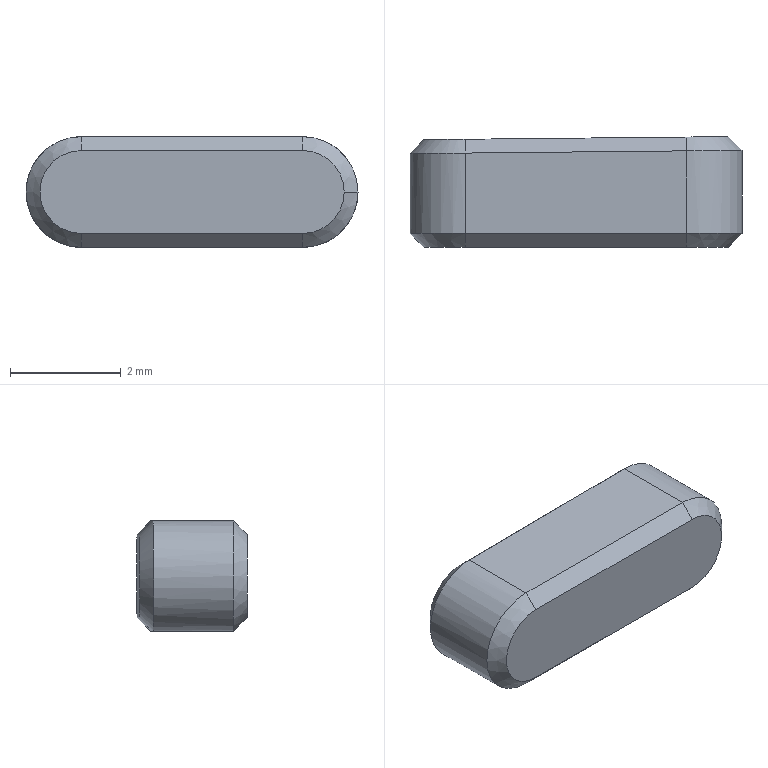Component | SolidWorks | taper keys for general use gb-2 | 1 solid | 16 faces | box 6 x 2 x 2 mm | volume 21 mm3 | plane 8 | cone 3 | cylinder 3 | spline 2 | commonest cylinder face diameters 2 x3
STEP:
#1=COLOUR_RGB('',0.7922,0.8196,0.9333);
#2=FILL_AREA_STYLE_COLOUR('',#1);
#3=FILL_AREA_STYLE('',(#2));
#4=SURFACE_STYLE_FILL_AREA(#3);
#5=SURFACE_SIDE_STYLE('',(#4));
#6=SURFACE_STYLE_USAGE(.BOTH.,#5);
#7=PRESENTATION_STYLE_ASSIGNMENT((#6));
#8=CARTESIAN_POINT('',(15.268,0.851,13.74));
#9=VERTEX_POINT('',#8);
#10=CARTESIAN_POINT('',(15.239,0.851,13.77));
#11=VERTEX_POINT('',#10);
#12=CARTESIAN_POINT('',(15.239,0.851,13.74));
#13=DIRECTION('',(-0.,-1.,0.));
#14=DIRECTION('',(1.,0.,0.));
#15=AXIS2_PLACEMENT_3D('',#12,#13,#14);
#16=CIRCLE('',#15,0.02953);
#17=EDGE_CURVE('',#9,#11,#16,.T.);
#18=ORIENTED_EDGE('',*,*,#17,.F.);
#19=CARTESIAN_POINT('',(15.278,0.8609,13.74));
#20=VERTEX_POINT('',#19);
#21=CARTESIAN_POINT('',(15.268,0.851,13.74));
#22=DIRECTION('',(0.7071,0.7071,-0.));
#23=VECTOR('',#22,39.37);
#24=LINE('',#21,#23);
#25=EDGE_CURVE('',#9,#20,#24,.T.);
#26=ORIENTED_EDGE('',*,*,#25,.T.);
#27=CARTESIAN_POINT('',(15.239,0.8609,13.78));
#28=VERTEX_POINT('',#27);
#29=CARTESIAN_POINT('',(15.239,0.8609,13.74));
#30=DIRECTION('',(0.,1.,-0.));
#31=DIRECTION('',(1.,0.,0.));
#32=AXIS2_PLACEMENT_3D('',#29,#30,#31);
#33=CIRCLE('',#32,0.03937);
#34=EDGE_CURVE('',#28,#20,#33,.T.);
#35=ORIENTED_EDGE('',*,*,#34,.F.);
#36=CARTESIAN_POINT('',(15.239,0.851,13.77));
#37=DIRECTION('',(-0.,0.7071,0.7071));
#38=VECTOR('',#37,39.37);
#39=LINE('',#36,#38);
#40=EDGE_CURVE('',#11,#28,#39,.T.);
#41=ORIENTED_EDGE('',*,*,#40,.F.);
#42=EDGE_LOOP('',(#18,#26,#35,#41));
#43=FACE_OUTER_BOUND('',#42,.T.);
#44=CARTESIAN_POINT('',(15.239,0.851,13.74));
#45=DIRECTION('',(0.,1.,-0.));
#46=DIRECTION('',(1.,0.,0.));
#47=AXIS2_PLACEMENT_3D('',#44,#45,#46);
#48=CONICAL_SURFACE('',#47,0.02953,0.7854);
#49=ADVANCED_FACE('',(#43),#48,.T.);
#50=ORIENTED_EDGE('',*,*,#34,.T.);
#51=CARTESIAN_POINT('',(15.278,0.9198,13.74));
#52=VERTEX_POINT('',#51);
#53=CARTESIAN_POINT('',(15.278,0.851,13.74));
#54=DIRECTION('',(0.,1.,-0.));
#55=VECTOR('',#54,39.37);
#56=LINE('',#53,#55);
#57=EDGE_CURVE('',#20,#52,#56,.T.);
#58=ORIENTED_EDGE('',*,*,#57,.T.);
#59=CARTESIAN_POINT('',(15.239,0.9195,13.78));
#60=VERTEX_POINT('',#59);
#61=CARTESIAN_POINT('',(15.278,0.9198,13.74));
#62=CARTESIAN_POINT('',(15.278,0.9198,13.744));
#63=CARTESIAN_POINT('',(15.277,0.9198,13.748));
#64=CARTESIAN_POINT('',(15.275,0.9198,13.756));
#65=CARTESIAN_POINT('',(15.273,0.9198,13.761));
#66=CARTESIAN_POINT('',(15.266,0.9197,13.769));
#67=CARTESIAN_POINT('',(15.262,0.9197,13.773));
#68=CARTESIAN_POINT('',(15.251,0.9196,13.778));
#69=CARTESIAN_POINT('',(15.245,0.9196,13.78));
#70=CARTESIAN_POINT('',(15.239,0.9195,13.78));
#71=B_SPLINE_CURVE_WITH_KNOTS('',3,(#61,#62,#63,#64,#65,#66,#67,#68,#69,#70),.UNSPECIFIED.,.F.,.F.,(4,2,2,2,4),(0.5,0.625,0.75,0.875,1.),.UNSPECIFIED.);
#72=EDGE_CURVE('',#52,#60,#71,.T.);
#73=ORIENTED_EDGE('',*,*,#72,.T.);
#74=CARTESIAN_POINT('',(15.239,0.851,13.78));
#75=DIRECTION('',(0.,1.,-0.));
#76=VECTOR('',#75,39.37);
#77=LINE('',#74,#76);
#78=EDGE_CURVE('',#28,#60,#77,.T.);
#79=ORIENTED_EDGE('',*,*,#78,.F.);
#80=EDGE_LOOP('',(#50,#58,#73,#79));
#81=FACE_OUTER_BOUND('',#80,.T.);
#82=CARTESIAN_POINT('',(15.239,0.851,13.74));
#83=DIRECTION('',(0.,1.,-0.));
#84=DIRECTION('',(1.,0.,0.));
#85=AXIS2_PLACEMENT_3D('',#82,#83,#84);
#86=CYLINDRICAL_SURFACE('',#85,0.03937);
#87=ADVANCED_FACE('',(#81),#86,.T.);
#88=ORIENTED_EDGE('',*,*,#57,.F.);
#89=CARTESIAN_POINT('',(15.239,0.8609,13.701));
#90=VERTEX_POINT('',#89);
#91=CARTESIAN_POINT('',(15.239,0.8609,13.74));
#92=DIRECTION('',(0.,1.,-0.));
#93=DIRECTION('',(1.,0.,0.));
#94=AXIS2_PLACEMENT_3D('',#91,#92,#93);
#95=CIRCLE('',#94,0.03937);
#96=EDGE_CURVE('',#20,#90,#95,.T.);
#97=ORIENTED_EDGE('',*,*,#96,.T.);
#98=CARTESIAN_POINT('',(15.239,0.9195,13.701));
#99=VERTEX_POINT('',#98);
#100=CARTESIAN_POINT('',(15.239,0.851,13.701));
#101=DIRECTION('',(0.,1.,-0.));
#102=VECTOR('',#101,39.37);
#103=LINE('',#100,#102);
#104=EDGE_CURVE('',#90,#99,#103,.T.);
#105=ORIENTED_EDGE('',*,*,#104,.T.);
#106=CARTESIAN_POINT('',(15.239,0.9195,13.701));
#107=CARTESIAN_POINT('',(15.245,0.9196,13.701));
#108=CARTESIAN_POINT('',(15.251,0.9196,13.702));
#109=CARTESIAN_POINT('',(15.262,0.9197,13.708));
#110=CARTESIAN_POINT('',(15.266,0.9197,13.711));
#111=CARTESIAN_POINT('',(15.273,0.9198,13.719));
#112=CARTESIAN_POINT('',(15.275,0.9198,13.724));
#113=CARTESIAN_POINT('',(15.277,0.9198,13.732));
#114=CARTESIAN_POINT('',(15.278,0.9198,13.736));
#115=CARTESIAN_POINT('',(15.278,0.9198,13.74));
#116=B_SPLINE_CURVE_WITH_KNOTS('',3,(#106,#107,#108,#109,#110,#111,#112,#113,#114,#115),.UNSPECIFIED.,.F.,.F.,(4,2,2,2,4),(0.,0.125,0.25,0.375,0.5),.UNSPECIFIED.);
#117=EDGE_CURVE('',#99,#52,#116,.T.);
#118=ORIENTED_EDGE('',*,*,#117,.T.);
#119=EDGE_LOOP('',(#88,#97,#105,#118));
#120=FACE_OUTER_BOUND('',#119,.T.);
#121=CARTESIAN_POINT('',(15.239,0.851,13.74));
#122=DIRECTION('',(0.,1.,-0.));
#123=DIRECTION('',(1.,0.,0.));
#124=AXIS2_PLACEMENT_3D('',#121,#122,#123);
#125=CYLINDRICAL_SURFACE('',#124,0.03937);
#126=ADVANCED_FACE('',(#120),#125,.T.);
#127=ORIENTED_EDGE('',*,*,#78,.T.);
#128=CARTESIAN_POINT('',(15.081,0.9179,13.78));
#129=VERTEX_POINT('',#128);
#130=CARTESIAN_POINT('',(15.081,0.9179,13.78));
#131=DIRECTION('',(-1.,-0.01,-0.));
#132=VECTOR('',#131,39.37);
#133=LINE('',#130,#132);
#134=EDGE_CURVE('',#60,#129,#133,.T.);
#135=ORIENTED_EDGE('',*,*,#134,.T.);
#136=CARTESIAN_POINT('',(15.081,0.8609,13.78));
#137=VERTEX_POINT('',#136);
#138=CARTESIAN_POINT('',(15.081,0.851,13.78));
#139=DIRECTION('',(0.,1.,-0.));
#140=VECTOR('',#139,39.37);
#141=LINE('',#138,#140);
#142=EDGE_CURVE('',#137,#129,#141,.T.);
#143=ORIENTED_EDGE('',*,*,#142,.F.);
#144=CARTESIAN_POINT('',(15.081,0.8609,13.78));
#145=DIRECTION('',(1.,0.,0.));
#146=VECTOR('',#145,39.37);
#147=LINE('',#144,#146);
#148=EDGE_CURVE('',#137,#28,#147,.T.);
#149=ORIENTED_EDGE('',*,*,#148,.T.);
#150=EDGE_LOOP('',(#127,#135,#143,#149));
#151=FACE_OUTER_BOUND('',#150,.T.);
#152=CARTESIAN_POINT('',(15.081,0.851,13.78));
#153=DIRECTION('',(0.,-0.,-1.));
#154=DIRECTION('',(1.,0.,0.));
#155=AXIS2_PLACEMENT_3D('',#152,#153,#154);
#156=PLANE('',#155);
#157=ADVANCED_FACE('',(#151),#156,.F.);
#158=ORIENTED_EDGE('',*,*,#142,.T.);
#159=CARTESIAN_POINT('',(15.081,0.9179,13.701));
#160=VERTEX_POINT('',#159);
#161=CARTESIAN_POINT('',(15.081,0.9179,13.78));
#162=CARTESIAN_POINT('',(15.071,0.9179,13.78));
#163=CARTESIAN_POINT('',(15.061,0.9178,13.775));
#164=CARTESIAN_POINT('',(15.046,0.9177,13.761));
#165=CARTESIAN_POINT('',(15.042,0.9177,13.75));
#166=CARTESIAN_POINT('',(15.042,0.9177,13.73));
#167=CARTESIAN_POINT('',(15.046,0.9177,13.72));
#168=CARTESIAN_POINT('',(15.061,0.9178,13.705));
#169=CARTESIAN_POINT('',(15.071,0.9179,13.701));
#170=CARTESIAN_POINT('',(15.081,0.9179,13.701));
#171=B_SPLINE_CURVE_WITH_KNOTS('',3,(#161,#162,#163,#164,#165,#166,#167,#168,#169,#170),.UNSPECIFIED.,.F.,.F.,(4,2,2,2,4),(0.,0.25,0.5,0.75,1.),.UNSPECIFIED.);
#172=EDGE_CURVE('',#129,#160,#171,.T.);
#173=ORIENTED_EDGE('',*,*,#172,.T.);
#174=CARTESIAN_POINT('',(15.081,0.8609,13.701));
#175=VERTEX_POINT('',#174);
#176=CARTESIAN_POINT('',(15.081,0.851,13.701));
#177=DIRECTION('',(0.,1.,-0.));
#178=VECTOR('',#177,39.37);
#179=LINE('',#176,#178);
#180=EDGE_CURVE('',#175,#160,#179,.T.);
#181=ORIENTED_EDGE('',*,*,#180,.F.);
#182=CARTESIAN_POINT('',(15.081,0.8609,13.74));
#183=DIRECTION('',(0.,1.,-0.));
#184=DIRECTION('',(1.,0.,0.));
#185=AXIS2_PLACEMENT_3D('',#182,#183,#184);
#186=CIRCLE('',#185,0.03937);
#187=EDGE_CURVE('',#175,#137,#186,.T.);
#188=ORIENTED_EDGE('',*,*,#187,.T.);
#189=EDGE_LOOP('',(#158,#173,#181,#188));
#190=FACE_OUTER_BOUND('',#189,.T.);
#191=CARTESIAN_POINT('',(15.081,0.851,13.74));
#192=DIRECTION('',(0.,1.,-0.));
#193=DIRECTION('',(1.,0.,0.));
#194=AXIS2_PLACEMENT_3D('',#191,#192,#193);
#195=CYLINDRICAL_SURFACE('',#194,0.03937);
#196=ADVANCED_FACE('',(#190),#195,.T.);
#197=ORIENTED_EDGE('',*,*,#180,.T.);
#198=CARTESIAN_POINT('',(15.238,0.9195,13.701));
#199=DIRECTION('',(1.,0.01,0.));
#200=VECTOR('',#199,39.37);
#201=LINE('',#198,#200);
#202=EDGE_CURVE('',#160,#99,#201,.T.);
#203=ORIENTED_EDGE('',*,*,#202,.T.);
#204=ORIENTED_EDGE('',*,*,#104,.F.);
#205=CARTESIAN_POINT('',(15.239,0.8609,13.701));
#206=DIRECTION('',(-1.,-0.,-0.));
#207=VECTOR('',#206,39.37);
#208=LINE('',#205,#207);
#209=EDGE_CURVE('',#90,#175,#208,.T.);
#210=ORIENTED_EDGE('',*,*,#209,.T.);
#211=EDGE_LOOP('',(#197,#203,#204,#210));
#212=FACE_OUTER_BOUND('',#211,.T.);
#213=CARTESIAN_POINT('',(15.239,0.851,13.701));
#214=DIRECTION('',(-0.,0.,1.));
#215=DIRECTION('',(0.,1.,-0.));
#216=AXIS2_PLACEMENT_3D('',#213,#214,#215);
#217=PLANE('',#216);
#218=ADVANCED_FACE('',(#212),#217,.F.);
#219=CARTESIAN_POINT('',(15.239,0.851,13.711));
#220=VERTEX_POINT('',#219);
#221=CARTESIAN_POINT('',(15.239,0.851,13.74));
#222=DIRECTION('',(-0.,-1.,0.));
#223=DIRECTION('',(1.,0.,0.));
#224=AXIS2_PLACEMENT_3D('',#221,#222,#223);
#225=CIRCLE('',#224,0.02953);
#226=EDGE_CURVE('',#220,#9,#225,.T.);
#227=ORIENTED_EDGE('',*,*,#226,.T.);
#228=ORIENTED_EDGE('',*,*,#17,.T.);
#229=CARTESIAN_POINT('',(15.081,0.851,13.77));
#230=VERTEX_POINT('',#229);
#231=CARTESIAN_POINT('',(15.239,0.851,13.77));
#232=DIRECTION('',(-1.,-0.,-0.));
#233=VECTOR('',#232,39.37);
#234=LINE('',#231,#233);
#235=EDGE_CURVE('',#11,#230,#234,.T.);
#236=ORIENTED_EDGE('',*,*,#235,.T.);
#237=CARTESIAN_POINT('',(15.081,0.851,13.711));
#238=VERTEX_POINT('',#237);
#239=CARTESIAN_POINT('',(15.081,0.851,13.74));
#240=DIRECTION('',(-0.,-1.,0.));
#241=DIRECTION('',(1.,0.,0.));
#242=AXIS2_PLACEMENT_3D('',#239,#240,#241);
#243=CIRCLE('',#242,0.02953);
#244=EDGE_CURVE('',#230,#238,#243,.T.);
#245=ORIENTED_EDGE('',*,*,#244,.T.);
#246=CARTESIAN_POINT('',(15.239,0.851,13.711));
#247=DIRECTION('',(1.,0.,0.));
#248=VECTOR('',#247,39.37);
#249=LINE('',#246,#248);
#250=EDGE_CURVE('',#238,#220,#249,.T.);
#251=ORIENTED_EDGE('',*,*,#250,.T.);
#252=EDGE_LOOP('',(#227,#228,#236,#245,#251));
#253=FACE_OUTER_BOUND('',#252,.T.);
#254=CARTESIAN_POINT('',(15.239,0.851,13.74));
#255=DIRECTION('',(0.,1.,-0.));
#256=DIRECTION('',(1.,0.,0.));
#257=AXIS2_PLACEMENT_3D('',#254,#255,#256);
#258=PLANE('',#257);
#259=ADVANCED_FACE('',(#253),#258,.F.);
#260=CARTESIAN_POINT('',(15.081,0.9278,13.711));
#261=VERTEX_POINT('',#260);
#262=CARTESIAN_POINT('',(15.081,0.9278,13.77));
#263=VERTEX_POINT('',#262);
#264=CARTESIAN_POINT('',(15.081,0.9278,13.711));
#265=CARTESIAN_POINT('',(15.073,0.9277,13.71));
#266=CARTESIAN_POINT('',(15.066,0.9276,13.713));
#267=CARTESIAN_POINT('',(15.055,0.9275,13.725));
#268=CARTESIAN_POINT('',(15.052,0.9275,13.732));
#269=CARTESIAN_POINT('',(15.052,0.9275,13.748));
#270=CARTESIAN_POINT('',(15.054,0.9275,13.755));
#271=CARTESIAN_POINT('',(15.066,0.9276,13.767));
#272=CARTESIAN_POINT('',(15.073,0.9277,13.77));
#273=CARTESIAN_POINT('',(15.081,0.9278,13.77));
#274=B_SPLINE_CURVE_WITH_KNOTS('',3,(#264,#265,#266,#267,#268,#269,#270,#271,#272,#273),.UNSPECIFIED.,.F.,.F.,(4,2,2,2,4),(0.,0.25,0.5,0.75,1.),.UNSPECIFIED.);
#275=EDGE_CURVE('',#261,#263,#274,.T.);
#276=ORIENTED_EDGE('',*,*,#275,.T.);
#277=CARTESIAN_POINT('',(15.239,0.9294,13.77));
#278=VERTEX_POINT('',#277);
#279=CARTESIAN_POINT('',(15.042,0.9274,13.77));
#280=DIRECTION('',(1.,0.01,0.));
#281=VECTOR('',#280,39.37);
#282=LINE('',#279,#281);
#283=EDGE_CURVE('',#263,#278,#282,.T.);
#284=ORIENTED_EDGE('',*,*,#283,.T.);
#285=CARTESIAN_POINT('',(15.239,0.9294,13.711));
#286=VERTEX_POINT('',#285);
#287=CARTESIAN_POINT('',(15.239,0.9294,13.77));
#288=CARTESIAN_POINT('',(15.246,0.9294,13.77));
#289=CARTESIAN_POINT('',(15.253,0.9295,13.767));
#290=CARTESIAN_POINT('',(15.265,0.9296,13.755));
#291=CARTESIAN_POINT('',(15.268,0.9297,13.748));
#292=CARTESIAN_POINT('',(15.268,0.9297,13.732));
#293=CARTESIAN_POINT('',(15.265,0.9296,13.725));
#294=CARTESIAN_POINT('',(15.253,0.9295,13.713));
#295=CARTESIAN_POINT('',(15.246,0.9294,13.71));
#296=CARTESIAN_POINT('',(15.239,0.9294,13.711));
#297=B_SPLINE_CURVE_WITH_KNOTS('',3,(#287,#288,#289,#290,#291,#292,#293,#294,#295,#296),.UNSPECIFIED.,.F.,.F.,(4,2,2,2,4),(0.,0.25,0.5,0.75,1.),.UNSPECIFIED.);
#298=EDGE_CURVE('',#278,#286,#297,.T.);
#299=ORIENTED_EDGE('',*,*,#298,.T.);
#300=CARTESIAN_POINT('',(15.042,0.9274,13.711));
#301=DIRECTION('',(-1.,-0.01,-0.));
#302=VECTOR('',#301,39.37);
#303=LINE('',#300,#302);
#304=EDGE_CURVE('',#286,#261,#303,.T.);
#305=ORIENTED_EDGE('',*,*,#304,.T.);
#306=EDGE_LOOP('',(#276,#284,#299,#305));
#307=FACE_OUTER_BOUND('',#306,.T.);
#308=CARTESIAN_POINT('',(15.042,0.9274,13.78));
#309=DIRECTION('',(0.01,-1.,0.));
#310=DIRECTION('',(-1.,-0.01,-0.));
#311=AXIS2_PLACEMENT_3D('',#308,#309,#310);
#312=PLANE('',#311);
#313=ADVANCED_FACE('',(#307),#312,.F.);
#314=CARTESIAN_POINT('',(15.081,0.9278,13.711));
#315=CARTESIAN_POINT('',(15.081,0.9179,13.701));
#316=B_SPLINE_CURVE_WITH_KNOTS('',1,(#314,#315),.UNSPECIFIED.,.F.,.F.,(2,2),(0.,1.),.UNSPECIFIED.);
#317=EDGE_CURVE('',#261,#160,#316,.T.);
#318=ORIENTED_EDGE('',*,*,#317,.F.);
#319=ORIENTED_EDGE('',*,*,#304,.F.);
#320=CARTESIAN_POINT('',(15.239,0.9195,13.701));
#321=CARTESIAN_POINT('',(15.239,0.9294,13.711));
#322=B_SPLINE_CURVE_WITH_KNOTS('',1,(#320,#321),.UNSPECIFIED.,.F.,.F.,(2,2),(0.,1.),.UNSPECIFIED.);
#323=EDGE_CURVE('',#99,#286,#322,.T.);
#324=ORIENTED_EDGE('',*,*,#323,.F.);
#325=ORIENTED_EDGE('',*,*,#202,.F.);
#326=EDGE_LOOP('',(#318,#319,#324,#325));
#327=FACE_OUTER_BOUND('',#326,.T.);
#328=CARTESIAN_POINT('',(15.042,0.9274,13.711));
#329=DIRECTION('',(0.007071,-0.7071,0.7071));
#330=DIRECTION('',(-0.,0.7071,0.7071));
#331=AXIS2_PLACEMENT_3D('',#328,#329,#330);
#332=PLANE('',#331);
#333=ADVANCED_FACE('',(#327),#332,.F.);
#334=ORIENTED_EDGE('',*,*,#323,.T.);
#335=ORIENTED_EDGE('',*,*,#298,.F.);
#336=CARTESIAN_POINT('',(15.239,0.9195,13.78));
#337=CARTESIAN_POINT('',(15.239,0.9228,13.776));
#338=CARTESIAN_POINT('',(15.239,0.9261,13.773));
#339=CARTESIAN_POINT('',(15.239,0.9294,13.77));
#340=B_SPLINE_CURVE_WITH_KNOTS('',3,(#336,#337,#338,#339),.UNSPECIFIED.,.F.,.F.,(4,4),(0.,1.),.UNSPECIFIED.);
#341=EDGE_CURVE('',#60,#278,#340,.T.);
#342=ORIENTED_EDGE('',*,*,#341,.F.);
#343=ORIENTED_EDGE('',*,*,#72,.F.);
#344=ORIENTED_EDGE('',*,*,#117,.F.);
#345=EDGE_LOOP('',(#334,#335,#342,#343,#344));
#346=FACE_OUTER_BOUND('',#345,.T.);
#347=CARTESIAN_POINT('',(15.239,0.9195,13.701));
#348=CARTESIAN_POINT('',(15.26,0.9197,13.7));
#349=CARTESIAN_POINT('',(15.278,0.9198,13.719));
#350=CARTESIAN_POINT('',(15.278,0.9198,13.761));
#351=CARTESIAN_POINT('',(15.26,0.9197,13.78));
#352=CARTESIAN_POINT('',(15.239,0.9195,13.78));
#353=CARTESIAN_POINT('',(15.239,0.9294,13.711));
#354=CARTESIAN_POINT('',(15.254,0.9295,13.71));
#355=CARTESIAN_POINT('',(15.268,0.9297,13.724));
#356=CARTESIAN_POINT('',(15.268,0.9297,13.756));
#357=CARTESIAN_POINT('',(15.254,0.9295,13.77));
#358=CARTESIAN_POINT('',(15.239,0.9294,13.77));
#359=B_SPLINE_SURFACE_WITH_KNOTS('',1,3,((#347,#348,#349,#350,#351,#352),(#353,#354,#355,#356,#357,#358)),.UNSPECIFIED.,.F.,.F.,.F.,(2,2),(4,2,4),(0.,1.),(4.712,6.283,7.854),.UNSPECIFIED.);
#360=ADVANCED_FACE('',(#346),#359,.T.);
#361=ORIENTED_EDGE('',*,*,#317,.T.);
#362=ORIENTED_EDGE('',*,*,#172,.F.);
#363=CARTESIAN_POINT('',(15.081,0.9278,13.77));
#364=CARTESIAN_POINT('',(15.081,0.9245,13.773));
#365=CARTESIAN_POINT('',(15.081,0.9212,13.776));
#366=CARTESIAN_POINT('',(15.081,0.9179,13.78));
#367=B_SPLINE_CURVE_WITH_KNOTS('',3,(#363,#364,#365,#366),.UNSPECIFIED.,.F.,.F.,(4,4),(0.,1.),.UNSPECIFIED.);
#368=EDGE_CURVE('',#263,#129,#367,.T.);
#369=ORIENTED_EDGE('',*,*,#368,.F.);
#370=ORIENTED_EDGE('',*,*,#275,.F.);
#371=EDGE_LOOP('',(#361,#362,#369,#370));
#372=FACE_OUTER_BOUND('',#371,.T.);
#373=CARTESIAN_POINT('',(15.081,0.9179,13.78));
#374=CARTESIAN_POINT('',(15.06,0.9178,13.78));
#375=CARTESIAN_POINT('',(15.042,0.9176,13.761));
#376=CARTESIAN_POINT('',(15.042,0.9176,13.719));
#377=CARTESIAN_POINT('',(15.06,0.9178,13.7));
#378=CARTESIAN_POINT('',(15.081,0.9179,13.701));
#379=CARTESIAN_POINT('',(15.081,0.9278,13.77));
#380=CARTESIAN_POINT('',(15.065,0.9276,13.77));
#381=CARTESIAN_POINT('',(15.052,0.9275,13.756));
#382=CARTESIAN_POINT('',(15.052,0.9275,13.724));
#383=CARTESIAN_POINT('',(15.065,0.9276,13.71));
#384=CARTESIAN_POINT('',(15.081,0.9278,13.711));
#385=B_SPLINE_SURFACE_WITH_KNOTS('',1,3,((#373,#374,#375,#376,#377,#378),(#379,#380,#381,#382,#383,#384)),.UNSPECIFIED.,.F.,.F.,.F.,(2,2),(4,2,4),(0.,1.),(1.571,3.142,4.712),.UNSPECIFIED.);
#386=ADVANCED_FACE('',(#372),#385,.T.);
#387=ORIENTED_EDGE('',*,*,#341,.T.);
#388=ORIENTED_EDGE('',*,*,#283,.F.);
#389=ORIENTED_EDGE('',*,*,#368,.T.);
#390=ORIENTED_EDGE('',*,*,#134,.F.);
#391=EDGE_LOOP('',(#387,#388,#389,#390));
#392=FACE_OUTER_BOUND('',#391,.T.);
#393=CARTESIAN_POINT('',(15.081,0.9179,13.78));
#394=DIRECTION('',(0.007071,-0.7071,-0.7071));
#395=DIRECTION('',(-0.,-0.7071,0.7071));
#396=AXIS2_PLACEMENT_3D('',#393,#394,#395);
#397=PLANE('',#396);
#398=ADVANCED_FACE('',(#392),#397,.F.);
#399=CARTESIAN_POINT('',(15.081,0.8609,13.701));
#400=DIRECTION('',(-0.,-0.7071,0.7071));
#401=VECTOR('',#400,39.37);
#402=LINE('',#399,#401);
#403=EDGE_CURVE('',#175,#238,#402,.T.);
#404=ORIENTED_EDGE('',*,*,#403,.F.);
#405=ORIENTED_EDGE('',*,*,#209,.F.);
#406=CARTESIAN_POINT('',(15.239,0.851,13.711));
#407=DIRECTION('',(0.,0.7071,-0.7071));
#408=VECTOR('',#407,39.37);
#409=LINE('',#406,#408);
#410=EDGE_CURVE('',#220,#90,#409,.T.);
#411=ORIENTED_EDGE('',*,*,#410,.F.);
#412=ORIENTED_EDGE('',*,*,#250,.F.);
#413=EDGE_LOOP('',(#404,#405,#411,#412));
#414=FACE_OUTER_BOUND('',#413,.T.);
#415=CARTESIAN_POINT('',(15.239,0.851,13.711));
#416=DIRECTION('',(-0.,0.7071,0.7071));
#417=DIRECTION('',(0.,0.7071,-0.7071));
#418=AXIS2_PLACEMENT_3D('',#415,#416,#417);
#419=PLANE('',#418);
#420=ADVANCED_FACE('',(#414),#419,.F.);
#421=ORIENTED_EDGE('',*,*,#25,.F.);
#422=ORIENTED_EDGE('',*,*,#226,.F.);
#423=ORIENTED_EDGE('',*,*,#410,.T.);
#424=ORIENTED_EDGE('',*,*,#96,.F.);
#425=EDGE_LOOP('',(#421,#422,#423,#424));
#426=FACE_OUTER_BOUND('',#425,.T.);
#427=CARTESIAN_POINT('',(15.239,0.851,13.74));
#428=DIRECTION('',(0.,1.,-0.));
#429=DIRECTION('',(1.,0.,0.));
#430=AXIS2_PLACEMENT_3D('',#427,#428,#429);
#431=CONICAL_SURFACE('',#430,0.02953,0.7854);
#432=ADVANCED_FACE('',(#426),#431,.T.);
#433=ORIENTED_EDGE('',*,*,#403,.T.);
#434=ORIENTED_EDGE('',*,*,#244,.F.);
#435=CARTESIAN_POINT('',(15.081,0.8609,13.78));
#436=DIRECTION('',(0.,-0.7071,-0.7071));
#437=VECTOR('',#436,39.37);
#438=LINE('',#435,#437);
#439=EDGE_CURVE('',#137,#230,#438,.T.);
#440=ORIENTED_EDGE('',*,*,#439,.F.);
#441=ORIENTED_EDGE('',*,*,#187,.F.);
#442=EDGE_LOOP('',(#433,#434,#440,#441));
#443=FACE_OUTER_BOUND('',#442,.T.);
#444=CARTESIAN_POINT('',(15.081,0.851,13.74));
#445=DIRECTION('',(0.,1.,-0.));
#446=DIRECTION('',(1.,0.,0.));
#447=AXIS2_PLACEMENT_3D('',#444,#445,#446);
#448=CONICAL_SURFACE('',#447,0.02953,0.7854);
#449=ADVANCED_FACE('',(#443),#448,.T.);
#450=ORIENTED_EDGE('',*,*,#40,.T.);
#451=ORIENTED_EDGE('',*,*,#148,.F.);
#452=ORIENTED_EDGE('',*,*,#439,.T.);
#453=ORIENTED_EDGE('',*,*,#235,.F.);
#454=EDGE_LOOP('',(#450,#451,#452,#453));
#455=FACE_OUTER_BOUND('',#454,.T.);
#456=CARTESIAN_POINT('',(15.239,0.851,13.77));
#457=DIRECTION('',(0.,0.7071,-0.7071));
#458=DIRECTION('',(0.,-0.7071,-0.7071));
#459=AXIS2_PLACEMENT_3D('',#456,#457,#458);
#460=PLANE('',#459);
#461=ADVANCED_FACE('',(#455),#460,.F.);
#462=CLOSED_SHELL('',(#49,#87,#126,#157,#196,#218,#259,#313,#333,#360,#386,#398,#420,#432,#449,#461));
#463=MANIFOLD_SOLID_BREP('',#462);
#464=STYLED_ITEM('',(#7),#463);
#465=PRESENTATION_LAYER_ASSIGNMENT('','',(#464));
#466=CARTESIAN_POINT('',(0.,0.,0.));
#467=DIRECTION('',(0.,0.,1.));
#468=DIRECTION('',(1.,0.,0.));
#469=AXIS2_PLACEMENT_3D('',#466,#467,#468);
#470=(LENGTH_UNIT()NAMED_UNIT(*)SI_UNIT($,.METRE.));
#471=LENGTH_MEASURE_WITH_UNIT(LENGTH_MEASURE(0.0254),#470);
#472=DIMENSIONAL_EXPONENTS(1.,0.,0.,0.,0.,0.,0.);
#473=(CONVERSION_BASED_UNIT('',#471)LENGTH_UNIT()NAMED_UNIT(#472));
#474=UNCERTAINTY_MEASURE_WITH_UNIT(LENGTH_MEASURE(0.00001),#473,'','');
#475=(NAMED_UNIT(*)PLANE_ANGLE_UNIT()SI_UNIT($,.RADIAN.));
#476=(NAMED_UNIT(*)SI_UNIT($,.STERADIAN.)SOLID_ANGLE_UNIT());
#477=(GEOMETRIC_REPRESENTATION_CONTEXT(3)GLOBAL_UNCERTAINTY_ASSIGNED_CONTEXT((#474))GLOBAL_UNIT_ASSIGNED_CONTEXT((#473,#475,#476))REPRESENTATION_CONTEXT('',''));
#478=ADVANCED_BREP_SHAPE_REPRESENTATION('',(#463,#469),#477);
#479=(LENGTH_UNIT()NAMED_UNIT(*)SI_UNIT($,.METRE.));
#480=LENGTH_MEASURE_WITH_UNIT(LENGTH_MEASURE(0.0254),#479);
#481=DIMENSIONAL_EXPONENTS(1.,0.,0.,0.,0.,0.,0.);
#482=(CONVERSION_BASED_UNIT('',#480)LENGTH_UNIT()NAMED_UNIT(#481));
#483=UNCERTAINTY_MEASURE_WITH_UNIT(LENGTH_MEASURE(0.00001),#482,'','');
#484=(NAMED_UNIT(*)PLANE_ANGLE_UNIT()SI_UNIT($,.RADIAN.));
#485=(NAMED_UNIT(*)SI_UNIT($,.STERADIAN.)SOLID_ANGLE_UNIT());
#486=(GEOMETRIC_REPRESENTATION_CONTEXT(3)GLOBAL_UNCERTAINTY_ASSIGNED_CONTEXT((#483))GLOBAL_UNIT_ASSIGNED_CONTEXT((#482,#484,#485))REPRESENTATION_CONTEXT('',''));
#487=MECHANICAL_DESIGN_GEOMETRIC_PRESENTATION_REPRESENTATION('',(#464),#486);